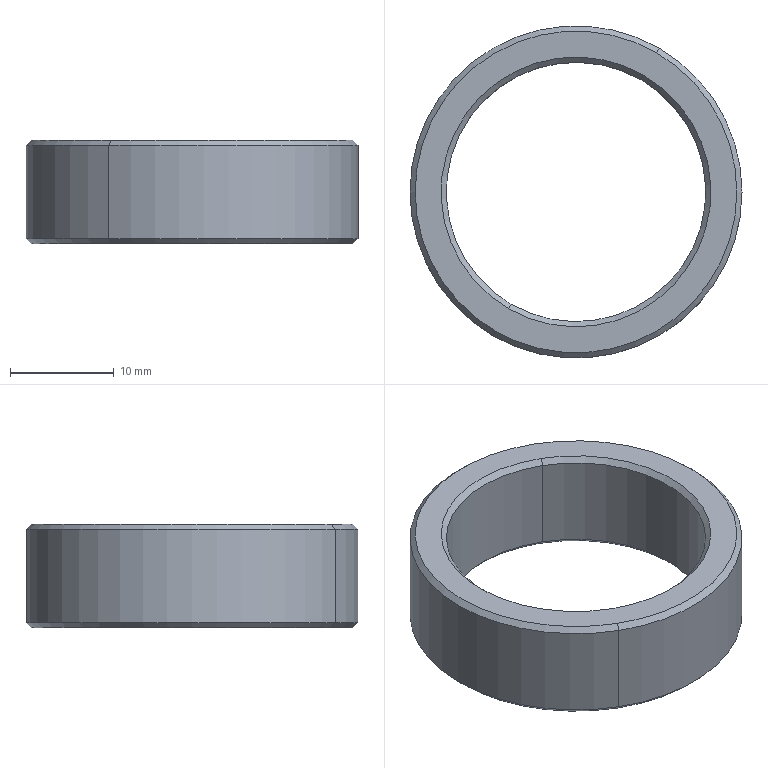Component | SolidWorks | Sleeve0-3 | 1 solid | 14 faces | box 32 x 32 x 10 mm | volume 3089 mm3 | cone 8 | cylinder 4 | plane 2 | commonest cylinder face diameters 32 x2 25 x2
build123d program:
from build123d import *


with BuildPart() as part:
    # Sketch1 → Revolve1 (revolve)
    with BuildSketch(Plane.XY, mode=Mode.PRIVATE) as revolve1_sk:
        Polygon((-4.5, 16), (4.5, 16), (5, 15.5), (5, 13), (4.5, 12.5), (-4.5, 12.5), (-5, 13), (-5, 15.5), align=None)
    revolve(revolve1_sk.sketch.rotate(Axis((-32.781, 0, 0), (1, 0, 0)), 90), axis=Axis((-32.781, 0, 0), (1, 0, 0)))


solid = part.part

# Placed as in the assembly
solid = solid.moved(Location((-15.093, -37.782, 261.455), (0, 90, 0)))
STEP:
#1=CARTESIAN_POINT('',(-0.2885,-0.9593,10.49));
#2=VERTEX_POINT('',#1);
#3=CARTESIAN_POINT('',(-0.8999,-2.016,10.49));
#4=VERTEX_POINT('',#3);
#5=CARTESIAN_POINT('',(-0.5942,-1.487,10.49));
#6=DIRECTION('',(-0.,0.,1.));
#7=DIRECTION('',(0.501,0.8655,0.));
#8=AXIS2_PLACEMENT_3D('',#5,#6,#7);
#9=CIRCLE('',#8,0.6102);
#10=EDGE_CURVE('',#2,#4,#9,.T.);
#11=ORIENTED_EDGE('',*,*,#10,.F.);
#12=CARTESIAN_POINT('',(-0.2786,-0.9423,10.471));
#13=VERTEX_POINT('',#12);
#14=CARTESIAN_POINT('',(-0.2786,-0.9423,10.471));
#15=DIRECTION('',(0.3542,0.612,-0.7071));
#16=VECTOR('',#15,39.37);
#17=LINE('',#14,#16);
#18=EDGE_CURVE('',#2,#13,#17,.T.);
#19=ORIENTED_EDGE('',*,*,#18,.T.);
#20=CARTESIAN_POINT('',(-0.9098,-2.033,10.471));
#21=VERTEX_POINT('',#20);
#22=CARTESIAN_POINT('',(-0.5942,-1.487,10.471));
#23=DIRECTION('',(-0.,0.,1.));
#24=DIRECTION('',(0.501,0.8655,0.));
#25=AXIS2_PLACEMENT_3D('',#22,#23,#24);
#26=CIRCLE('',#25,0.6299);
#27=EDGE_CURVE('',#13,#21,#26,.T.);
#28=ORIENTED_EDGE('',*,*,#27,.T.);
#29=CARTESIAN_POINT('',(-0.9098,-2.033,10.471));
#30=DIRECTION('',(-0.3542,-0.612,-0.7071));
#31=VECTOR('',#30,39.37);
#32=LINE('',#29,#31);
#33=EDGE_CURVE('',#4,#21,#32,.T.);
#34=ORIENTED_EDGE('',*,*,#33,.F.);
#35=EDGE_LOOP('',(#11,#19,#28,#34));
#36=FACE_OUTER_BOUND('',#35,.T.);
#37=CARTESIAN_POINT('',(-0.5942,-1.487,10.471));
#38=DIRECTION('',(0.,-0.,-1.));
#39=DIRECTION('',(-0.501,-0.8655,0.));
#40=AXIS2_PLACEMENT_3D('',#37,#38,#39);
#41=CONICAL_SURFACE('',#40,0.6299,0.7854);
#42=ADVANCED_FACE('',(#36),#41,.T.);
#43=CARTESIAN_POINT('',(-0.2786,-0.9423,10.116));
#44=VERTEX_POINT('',#43);
#45=CARTESIAN_POINT('',(-0.9098,-2.033,10.116));
#46=VERTEX_POINT('',#45);
#47=CARTESIAN_POINT('',(-0.5942,-1.487,10.116));
#48=DIRECTION('',(-0.,0.,1.));
#49=DIRECTION('',(0.501,0.8655,0.));
#50=AXIS2_PLACEMENT_3D('',#47,#48,#49);
#51=CIRCLE('',#50,0.6299);
#52=EDGE_CURVE('',#44,#46,#51,.T.);
#53=ORIENTED_EDGE('',*,*,#52,.T.);
#54=CARTESIAN_POINT('',(-0.9098,-2.033,11.584));
#55=DIRECTION('',(-0.,0.,1.));
#56=VECTOR('',#55,39.37);
#57=LINE('',#54,#56);
#58=EDGE_CURVE('',#46,#21,#57,.T.);
#59=ORIENTED_EDGE('',*,*,#58,.T.);
#60=ORIENTED_EDGE('',*,*,#27,.F.);
#61=CARTESIAN_POINT('',(-0.2786,-0.9423,11.584));
#62=DIRECTION('',(-0.,0.,1.));
#63=VECTOR('',#62,39.37);
#64=LINE('',#61,#63);
#65=EDGE_CURVE('',#44,#13,#64,.T.);
#66=ORIENTED_EDGE('',*,*,#65,.F.);
#67=EDGE_LOOP('',(#53,#59,#60,#66));
#68=FACE_OUTER_BOUND('',#67,.T.);
#69=CARTESIAN_POINT('',(-0.5942,-1.487,11.584));
#70=DIRECTION('',(-0.,0.,1.));
#71=DIRECTION('',(0.501,0.8655,0.));
#72=AXIS2_PLACEMENT_3D('',#69,#70,#71);
#73=CYLINDRICAL_SURFACE('',#72,0.6299);
#74=ADVANCED_FACE('',(#68),#73,.T.);
#75=CARTESIAN_POINT('',(-0.2885,-0.9593,10.097));
#76=VERTEX_POINT('',#75);
#77=CARTESIAN_POINT('',(-0.8999,-2.016,10.097));
#78=VERTEX_POINT('',#77);
#79=CARTESIAN_POINT('',(-0.5942,-1.487,10.097));
#80=DIRECTION('',(-0.,0.,1.));
#81=DIRECTION('',(0.501,0.8655,0.));
#82=AXIS2_PLACEMENT_3D('',#79,#80,#81);
#83=CIRCLE('',#82,0.6102);
#84=EDGE_CURVE('',#76,#78,#83,.T.);
#85=ORIENTED_EDGE('',*,*,#84,.T.);
#86=CARTESIAN_POINT('',(-0.8999,-2.016,10.097));
#87=DIRECTION('',(-0.3542,-0.612,0.7071));
#88=VECTOR('',#87,39.37);
#89=LINE('',#86,#88);
#90=EDGE_CURVE('',#78,#46,#89,.T.);
#91=ORIENTED_EDGE('',*,*,#90,.T.);
#92=ORIENTED_EDGE('',*,*,#52,.F.);
#93=CARTESIAN_POINT('',(-0.2885,-0.9593,10.097));
#94=DIRECTION('',(0.3542,0.612,0.7071));
#95=VECTOR('',#94,39.37);
#96=LINE('',#93,#95);
#97=EDGE_CURVE('',#76,#44,#96,.T.);
#98=ORIENTED_EDGE('',*,*,#97,.F.);
#99=EDGE_LOOP('',(#85,#91,#92,#98));
#100=FACE_OUTER_BOUND('',#99,.T.);
#101=CARTESIAN_POINT('',(-0.5942,-1.487,10.097));
#102=DIRECTION('',(-0.,0.,1.));
#103=DIRECTION('',(0.501,0.8655,0.));
#104=AXIS2_PLACEMENT_3D('',#101,#102,#103);
#105=CONICAL_SURFACE('',#104,0.6102,0.7854);
#106=ADVANCED_FACE('',(#100),#105,.T.);
#107=CARTESIAN_POINT('',(-0.8408,-1.913,10.116));
#108=VERTEX_POINT('',#107);
#109=CARTESIAN_POINT('',(-0.3477,-1.062,10.116));
#110=VERTEX_POINT('',#109);
#111=CARTESIAN_POINT('',(-0.5942,-1.487,10.116));
#112=DIRECTION('',(-0.,0.,1.));
#113=DIRECTION('',(0.501,0.8655,0.));
#114=AXIS2_PLACEMENT_3D('',#111,#112,#113);
#115=CIRCLE('',#114,0.4921);
#116=EDGE_CURVE('',#108,#110,#115,.T.);
#117=ORIENTED_EDGE('',*,*,#116,.T.);
#118=CARTESIAN_POINT('',(-0.3378,-1.045,10.097));
#119=VERTEX_POINT('',#118);
#120=CARTESIAN_POINT('',(-0.3477,-1.062,10.116));
#121=DIRECTION('',(0.3542,0.612,-0.7071));
#122=VECTOR('',#121,39.37);
#123=LINE('',#120,#122);
#124=EDGE_CURVE('',#110,#119,#123,.T.);
#125=ORIENTED_EDGE('',*,*,#124,.T.);
#126=CARTESIAN_POINT('',(-0.8506,-1.93,10.097));
#127=VERTEX_POINT('',#126);
#128=CARTESIAN_POINT('',(-0.5942,-1.487,10.097));
#129=DIRECTION('',(-0.,0.,1.));
#130=DIRECTION('',(0.501,0.8655,0.));
#131=AXIS2_PLACEMENT_3D('',#128,#129,#130);
#132=CIRCLE('',#131,0.5118);
#133=EDGE_CURVE('',#127,#119,#132,.T.);
#134=ORIENTED_EDGE('',*,*,#133,.F.);
#135=CARTESIAN_POINT('',(-0.8408,-1.913,10.116));
#136=DIRECTION('',(-0.3542,-0.612,-0.7071));
#137=VECTOR('',#136,39.37);
#138=LINE('',#135,#137);
#139=EDGE_CURVE('',#108,#127,#138,.T.);
#140=ORIENTED_EDGE('',*,*,#139,.F.);
#141=EDGE_LOOP('',(#117,#125,#134,#140));
#142=FACE_OUTER_BOUND('',#141,.T.);
#143=CARTESIAN_POINT('',(-0.5942,-1.487,10.116));
#144=DIRECTION('',(0.,-0.,-1.));
#145=DIRECTION('',(-0.501,-0.8655,0.));
#146=AXIS2_PLACEMENT_3D('',#143,#144,#145);
#147=CONICAL_SURFACE('',#146,0.4921,0.7854);
#148=ADVANCED_FACE('',(#142),#147,.F.);
#149=ORIENTED_EDGE('',*,*,#116,.F.);
#150=CARTESIAN_POINT('',(-0.8408,-1.913,10.471));
#151=VERTEX_POINT('',#150);
#152=CARTESIAN_POINT('',(-0.8408,-1.913,11.584));
#153=DIRECTION('',(-0.,0.,1.));
#154=VECTOR('',#153,39.37);
#155=LINE('',#152,#154);
#156=EDGE_CURVE('',#108,#151,#155,.T.);
#157=ORIENTED_EDGE('',*,*,#156,.T.);
#158=CARTESIAN_POINT('',(-0.3477,-1.062,10.471));
#159=VERTEX_POINT('',#158);
#160=CARTESIAN_POINT('',(-0.5942,-1.487,10.471));
#161=DIRECTION('',(-0.,0.,1.));
#162=DIRECTION('',(0.501,0.8655,0.));
#163=AXIS2_PLACEMENT_3D('',#160,#161,#162);
#164=CIRCLE('',#163,0.4921);
#165=EDGE_CURVE('',#151,#159,#164,.T.);
#166=ORIENTED_EDGE('',*,*,#165,.T.);
#167=CARTESIAN_POINT('',(-0.3477,-1.062,11.584));
#168=DIRECTION('',(-0.,0.,1.));
#169=VECTOR('',#168,39.37);
#170=LINE('',#167,#169);
#171=EDGE_CURVE('',#110,#159,#170,.T.);
#172=ORIENTED_EDGE('',*,*,#171,.F.);
#173=EDGE_LOOP('',(#149,#157,#166,#172));
#174=FACE_OUTER_BOUND('',#173,.T.);
#175=CARTESIAN_POINT('',(-0.5942,-1.487,11.584));
#176=DIRECTION('',(-0.,0.,1.));
#177=DIRECTION('',(0.501,0.8655,0.));
#178=AXIS2_PLACEMENT_3D('',#175,#176,#177);
#179=CYLINDRICAL_SURFACE('',#178,0.4921);
#180=ADVANCED_FACE('',(#174),#179,.F.);
#181=ORIENTED_EDGE('',*,*,#165,.F.);
#182=CARTESIAN_POINT('',(-0.8506,-1.93,10.49));
#183=VERTEX_POINT('',#182);
#184=CARTESIAN_POINT('',(-0.8506,-1.93,10.49));
#185=DIRECTION('',(-0.3542,-0.612,0.7071));
#186=VECTOR('',#185,39.37);
#187=LINE('',#184,#186);
#188=EDGE_CURVE('',#151,#183,#187,.T.);
#189=ORIENTED_EDGE('',*,*,#188,.T.);
#190=CARTESIAN_POINT('',(-0.3378,-1.045,10.49));
#191=VERTEX_POINT('',#190);
#192=CARTESIAN_POINT('',(-0.5942,-1.487,10.49));
#193=DIRECTION('',(-0.,0.,1.));
#194=DIRECTION('',(0.501,0.8655,0.));
#195=AXIS2_PLACEMENT_3D('',#192,#193,#194);
#196=CIRCLE('',#195,0.5118);
#197=EDGE_CURVE('',#183,#191,#196,.T.);
#198=ORIENTED_EDGE('',*,*,#197,.T.);
#199=CARTESIAN_POINT('',(-0.3378,-1.045,10.49));
#200=DIRECTION('',(0.3542,0.612,0.7071));
#201=VECTOR('',#200,39.37);
#202=LINE('',#199,#201);
#203=EDGE_CURVE('',#159,#191,#202,.T.);
#204=ORIENTED_EDGE('',*,*,#203,.F.);
#205=EDGE_LOOP('',(#181,#189,#198,#204));
#206=FACE_OUTER_BOUND('',#205,.T.);
#207=CARTESIAN_POINT('',(-0.5942,-1.487,10.49));
#208=DIRECTION('',(-0.,0.,1.));
#209=DIRECTION('',(0.501,0.8655,0.));
#210=AXIS2_PLACEMENT_3D('',#207,#208,#209);
#211=CONICAL_SURFACE('',#210,0.5118,0.7854);
#212=ADVANCED_FACE('',(#206),#211,.F.);
#213=ORIENTED_EDGE('',*,*,#188,.F.);
#214=CARTESIAN_POINT('',(-0.5942,-1.487,10.471));
#215=DIRECTION('',(-0.,0.,1.));
#216=DIRECTION('',(0.501,0.8655,0.));
#217=AXIS2_PLACEMENT_3D('',#214,#215,#216);
#218=CIRCLE('',#217,0.4921);
#219=EDGE_CURVE('',#159,#151,#218,.T.);
#220=ORIENTED_EDGE('',*,*,#219,.F.);
#221=ORIENTED_EDGE('',*,*,#203,.T.);
#222=CARTESIAN_POINT('',(-0.5942,-1.487,10.49));
#223=DIRECTION('',(-0.,0.,1.));
#224=DIRECTION('',(0.501,0.8655,0.));
#225=AXIS2_PLACEMENT_3D('',#222,#223,#224);
#226=CIRCLE('',#225,0.5118);
#227=EDGE_CURVE('',#191,#183,#226,.T.);
#228=ORIENTED_EDGE('',*,*,#227,.T.);
#229=EDGE_LOOP('',(#213,#220,#221,#228));
#230=FACE_OUTER_BOUND('',#229,.T.);
#231=CARTESIAN_POINT('',(-0.5942,-1.487,10.49));
#232=DIRECTION('',(-0.,0.,1.));
#233=DIRECTION('',(0.501,0.8655,0.));
#234=AXIS2_PLACEMENT_3D('',#231,#232,#233);
#235=CONICAL_SURFACE('',#234,0.5118,0.7854);
#236=ADVANCED_FACE('',(#230),#235,.F.);
#237=ORIENTED_EDGE('',*,*,#156,.F.);
#238=CARTESIAN_POINT('',(-0.5942,-1.487,10.116));
#239=DIRECTION('',(-0.,0.,1.));
#240=DIRECTION('',(0.501,0.8655,0.));
#241=AXIS2_PLACEMENT_3D('',#238,#239,#240);
#242=CIRCLE('',#241,0.4921);
#243=EDGE_CURVE('',#110,#108,#242,.T.);
#244=ORIENTED_EDGE('',*,*,#243,.F.);
#245=ORIENTED_EDGE('',*,*,#171,.T.);
#246=ORIENTED_EDGE('',*,*,#219,.T.);
#247=EDGE_LOOP('',(#237,#244,#245,#246));
#248=FACE_OUTER_BOUND('',#247,.T.);
#249=CARTESIAN_POINT('',(-0.5942,-1.487,11.584));
#250=DIRECTION('',(-0.,0.,1.));
#251=DIRECTION('',(0.501,0.8655,0.));
#252=AXIS2_PLACEMENT_3D('',#249,#250,#251);
#253=CYLINDRICAL_SURFACE('',#252,0.4921);
#254=ADVANCED_FACE('',(#248),#253,.F.);
#255=ORIENTED_EDGE('',*,*,#124,.F.);
#256=ORIENTED_EDGE('',*,*,#243,.T.);
#257=ORIENTED_EDGE('',*,*,#139,.T.);
#258=CARTESIAN_POINT('',(-0.5942,-1.487,10.097));
#259=DIRECTION('',(-0.,0.,1.));
#260=DIRECTION('',(0.501,0.8655,0.));
#261=AXIS2_PLACEMENT_3D('',#258,#259,#260);
#262=CIRCLE('',#261,0.5118);
#263=EDGE_CURVE('',#119,#127,#262,.T.);
#264=ORIENTED_EDGE('',*,*,#263,.F.);
#265=EDGE_LOOP('',(#255,#256,#257,#264));
#266=FACE_OUTER_BOUND('',#265,.T.);
#267=CARTESIAN_POINT('',(-0.5942,-1.487,10.116));
#268=DIRECTION('',(0.,-0.,-1.));
#269=DIRECTION('',(-0.501,-0.8655,0.));
#270=AXIS2_PLACEMENT_3D('',#267,#268,#269);
#271=CONICAL_SURFACE('',#270,0.4921,0.7854);
#272=ADVANCED_FACE('',(#266),#271,.F.);
#273=ORIENTED_EDGE('',*,*,#84,.F.);
#274=CARTESIAN_POINT('',(-0.5942,-1.487,10.097));
#275=DIRECTION('',(-0.,0.,1.));
#276=DIRECTION('',(0.501,0.8655,0.));
#277=AXIS2_PLACEMENT_3D('',#274,#275,#276);
#278=CIRCLE('',#277,0.6102);
#279=EDGE_CURVE('',#78,#76,#278,.T.);
#280=ORIENTED_EDGE('',*,*,#279,.F.);
#281=EDGE_LOOP('',(#273,#280));
#282=FACE_OUTER_BOUND('',#281,.T.);
#283=ORIENTED_EDGE('',*,*,#133,.T.);
#284=ORIENTED_EDGE('',*,*,#263,.T.);
#285=EDGE_LOOP('',(#283,#284));
#286=FACE_BOUND('',#285,.T.);
#287=CARTESIAN_POINT('',(-1.122,-1.182,10.097));
#288=DIRECTION('',(-0.,0.,1.));
#289=DIRECTION('',(0.501,0.8655,-0.));
#290=AXIS2_PLACEMENT_3D('',#287,#288,#289);
#291=PLANE('',#290);
#292=ADVANCED_FACE('',(#282,#286),#291,.F.);
#293=ORIENTED_EDGE('',*,*,#90,.F.);
#294=ORIENTED_EDGE('',*,*,#279,.T.);
#295=ORIENTED_EDGE('',*,*,#97,.T.);
#296=CARTESIAN_POINT('',(-0.5942,-1.487,10.116));
#297=DIRECTION('',(-0.,0.,1.));
#298=DIRECTION('',(0.501,0.8655,0.));
#299=AXIS2_PLACEMENT_3D('',#296,#297,#298);
#300=CIRCLE('',#299,0.6299);
#301=EDGE_CURVE('',#46,#44,#300,.T.);
#302=ORIENTED_EDGE('',*,*,#301,.F.);
#303=EDGE_LOOP('',(#293,#294,#295,#302));
#304=FACE_OUTER_BOUND('',#303,.T.);
#305=CARTESIAN_POINT('',(-0.5942,-1.487,10.097));
#306=DIRECTION('',(-0.,0.,1.));
#307=DIRECTION('',(0.501,0.8655,0.));
#308=AXIS2_PLACEMENT_3D('',#305,#306,#307);
#309=CONICAL_SURFACE('',#308,0.6102,0.7854);
#310=ADVANCED_FACE('',(#304),#309,.T.);
#311=ORIENTED_EDGE('',*,*,#58,.F.);
#312=ORIENTED_EDGE('',*,*,#301,.T.);
#313=ORIENTED_EDGE('',*,*,#65,.T.);
#314=CARTESIAN_POINT('',(-0.5942,-1.487,10.471));
#315=DIRECTION('',(-0.,0.,1.));
#316=DIRECTION('',(0.501,0.8655,0.));
#317=AXIS2_PLACEMENT_3D('',#314,#315,#316);
#318=CIRCLE('',#317,0.6299);
#319=EDGE_CURVE('',#21,#13,#318,.T.);
#320=ORIENTED_EDGE('',*,*,#319,.F.);
#321=EDGE_LOOP('',(#311,#312,#313,#320));
#322=FACE_OUTER_BOUND('',#321,.T.);
#323=CARTESIAN_POINT('',(-0.5942,-1.487,11.584));
#324=DIRECTION('',(-0.,0.,1.));
#325=DIRECTION('',(0.501,0.8655,0.));
#326=AXIS2_PLACEMENT_3D('',#323,#324,#325);
#327=CYLINDRICAL_SURFACE('',#326,0.6299);
#328=ADVANCED_FACE('',(#322),#327,.T.);
#329=ORIENTED_EDGE('',*,*,#18,.F.);
#330=CARTESIAN_POINT('',(-0.5942,-1.487,10.49));
#331=DIRECTION('',(-0.,0.,1.));
#332=DIRECTION('',(0.501,0.8655,0.));
#333=AXIS2_PLACEMENT_3D('',#330,#331,#332);
#334=CIRCLE('',#333,0.6102);
#335=EDGE_CURVE('',#4,#2,#334,.T.);
#336=ORIENTED_EDGE('',*,*,#335,.F.);
#337=ORIENTED_EDGE('',*,*,#33,.T.);
#338=ORIENTED_EDGE('',*,*,#319,.T.);
#339=EDGE_LOOP('',(#329,#336,#337,#338));
#340=FACE_OUTER_BOUND('',#339,.T.);
#341=CARTESIAN_POINT('',(-0.5942,-1.487,10.471));
#342=DIRECTION('',(0.,-0.,-1.));
#343=DIRECTION('',(-0.501,-0.8655,0.));
#344=AXIS2_PLACEMENT_3D('',#341,#342,#343);
#345=CONICAL_SURFACE('',#344,0.6299,0.7854);
#346=ADVANCED_FACE('',(#340),#345,.T.);
#347=ORIENTED_EDGE('',*,*,#227,.F.);
#348=ORIENTED_EDGE('',*,*,#197,.F.);
#349=EDGE_LOOP('',(#347,#348));
#350=FACE_BOUND('',#349,.T.);
#351=ORIENTED_EDGE('',*,*,#335,.T.);
#352=ORIENTED_EDGE('',*,*,#10,.T.);
#353=EDGE_LOOP('',(#351,#352));
#354=FACE_OUTER_BOUND('',#353,.T.);
#355=CARTESIAN_POINT('',(-1.122,-1.182,10.49));
#356=DIRECTION('',(0.,-0.,-1.));
#357=DIRECTION('',(-0.501,-0.8655,0.));
#358=AXIS2_PLACEMENT_3D('',#355,#356,#357);
#359=PLANE('',#358);
#360=ADVANCED_FACE('',(#350,#354),#359,.F.);
#361=CLOSED_SHELL('',(#42,#74,#106,#148,#180,#212,#236,#254,#272,#292,#310,#328,#346,#360));
#362=MANIFOLD_SOLID_BREP('',#361);
#363=CARTESIAN_POINT('',(0.,0.,0.));
#364=DIRECTION('',(0.,0.,1.));
#365=DIRECTION('',(1.,0.,0.));
#366=AXIS2_PLACEMENT_3D('',#363,#364,#365);
#367=(LENGTH_UNIT()NAMED_UNIT(*)SI_UNIT($,.METRE.));
#368=LENGTH_MEASURE_WITH_UNIT(LENGTH_MEASURE(0.0254),#367);
#369=DIMENSIONAL_EXPONENTS(1.,0.,0.,0.,0.,0.,0.);
#370=(CONVERSION_BASED_UNIT('',#368)LENGTH_UNIT()NAMED_UNIT(#369));
#371=UNCERTAINTY_MEASURE_WITH_UNIT(LENGTH_MEASURE(0.00001),#370,'','');
#372=(NAMED_UNIT(*)PLANE_ANGLE_UNIT()SI_UNIT($,.RADIAN.));
#373=(NAMED_UNIT(*)SI_UNIT($,.STERADIAN.)SOLID_ANGLE_UNIT());
#374=(GEOMETRIC_REPRESENTATION_CONTEXT(3)GLOBAL_UNCERTAINTY_ASSIGNED_CONTEXT((#371))GLOBAL_UNIT_ASSIGNED_CONTEXT((#370,#372,#373))REPRESENTATION_CONTEXT('',''));
#375=ADVANCED_BREP_SHAPE_REPRESENTATION('',(#362,#366),#374);
#376=COLOUR_RGB('',0.7922,0.8196,0.9333);
#377=FILL_AREA_STYLE_COLOUR('',#376);
#378=FILL_AREA_STYLE('',(#377));
#379=SURFACE_STYLE_FILL_AREA(#378);
#380=SURFACE_SIDE_STYLE('',(#379));
#381=SURFACE_STYLE_USAGE(.BOTH.,#380);
#382=PRESENTATION_STYLE_ASSIGNMENT((#381));
#383=STYLED_ITEM('',(#382),#362);
#384=PRESENTATION_LAYER_ASSIGNMENT('','',(#383));
#385=(LENGTH_UNIT()NAMED_UNIT(*)SI_UNIT($,.METRE.));
#386=LENGTH_MEASURE_WITH_UNIT(LENGTH_MEASURE(0.0254),#385);
#387=DIMENSIONAL_EXPONENTS(1.,0.,0.,0.,0.,0.,0.);
#388=(CONVERSION_BASED_UNIT('',#386)LENGTH_UNIT()NAMED_UNIT(#387));
#389=UNCERTAINTY_MEASURE_WITH_UNIT(LENGTH_MEASURE(0.00001),#388,'','');
#390=(NAMED_UNIT(*)PLANE_ANGLE_UNIT()SI_UNIT($,.RADIAN.));
#391=(NAMED_UNIT(*)SI_UNIT($,.STERADIAN.)SOLID_ANGLE_UNIT());
#392=(GEOMETRIC_REPRESENTATION_CONTEXT(3)GLOBAL_UNCERTAINTY_ASSIGNED_CONTEXT((#389))GLOBAL_UNIT_ASSIGNED_CONTEXT((#388,#390,#391))REPRESENTATION_CONTEXT('',''));
#393=MECHANICAL_DESIGN_GEOMETRIC_PRESENTATION_REPRESENTATION('',(#383),#392);